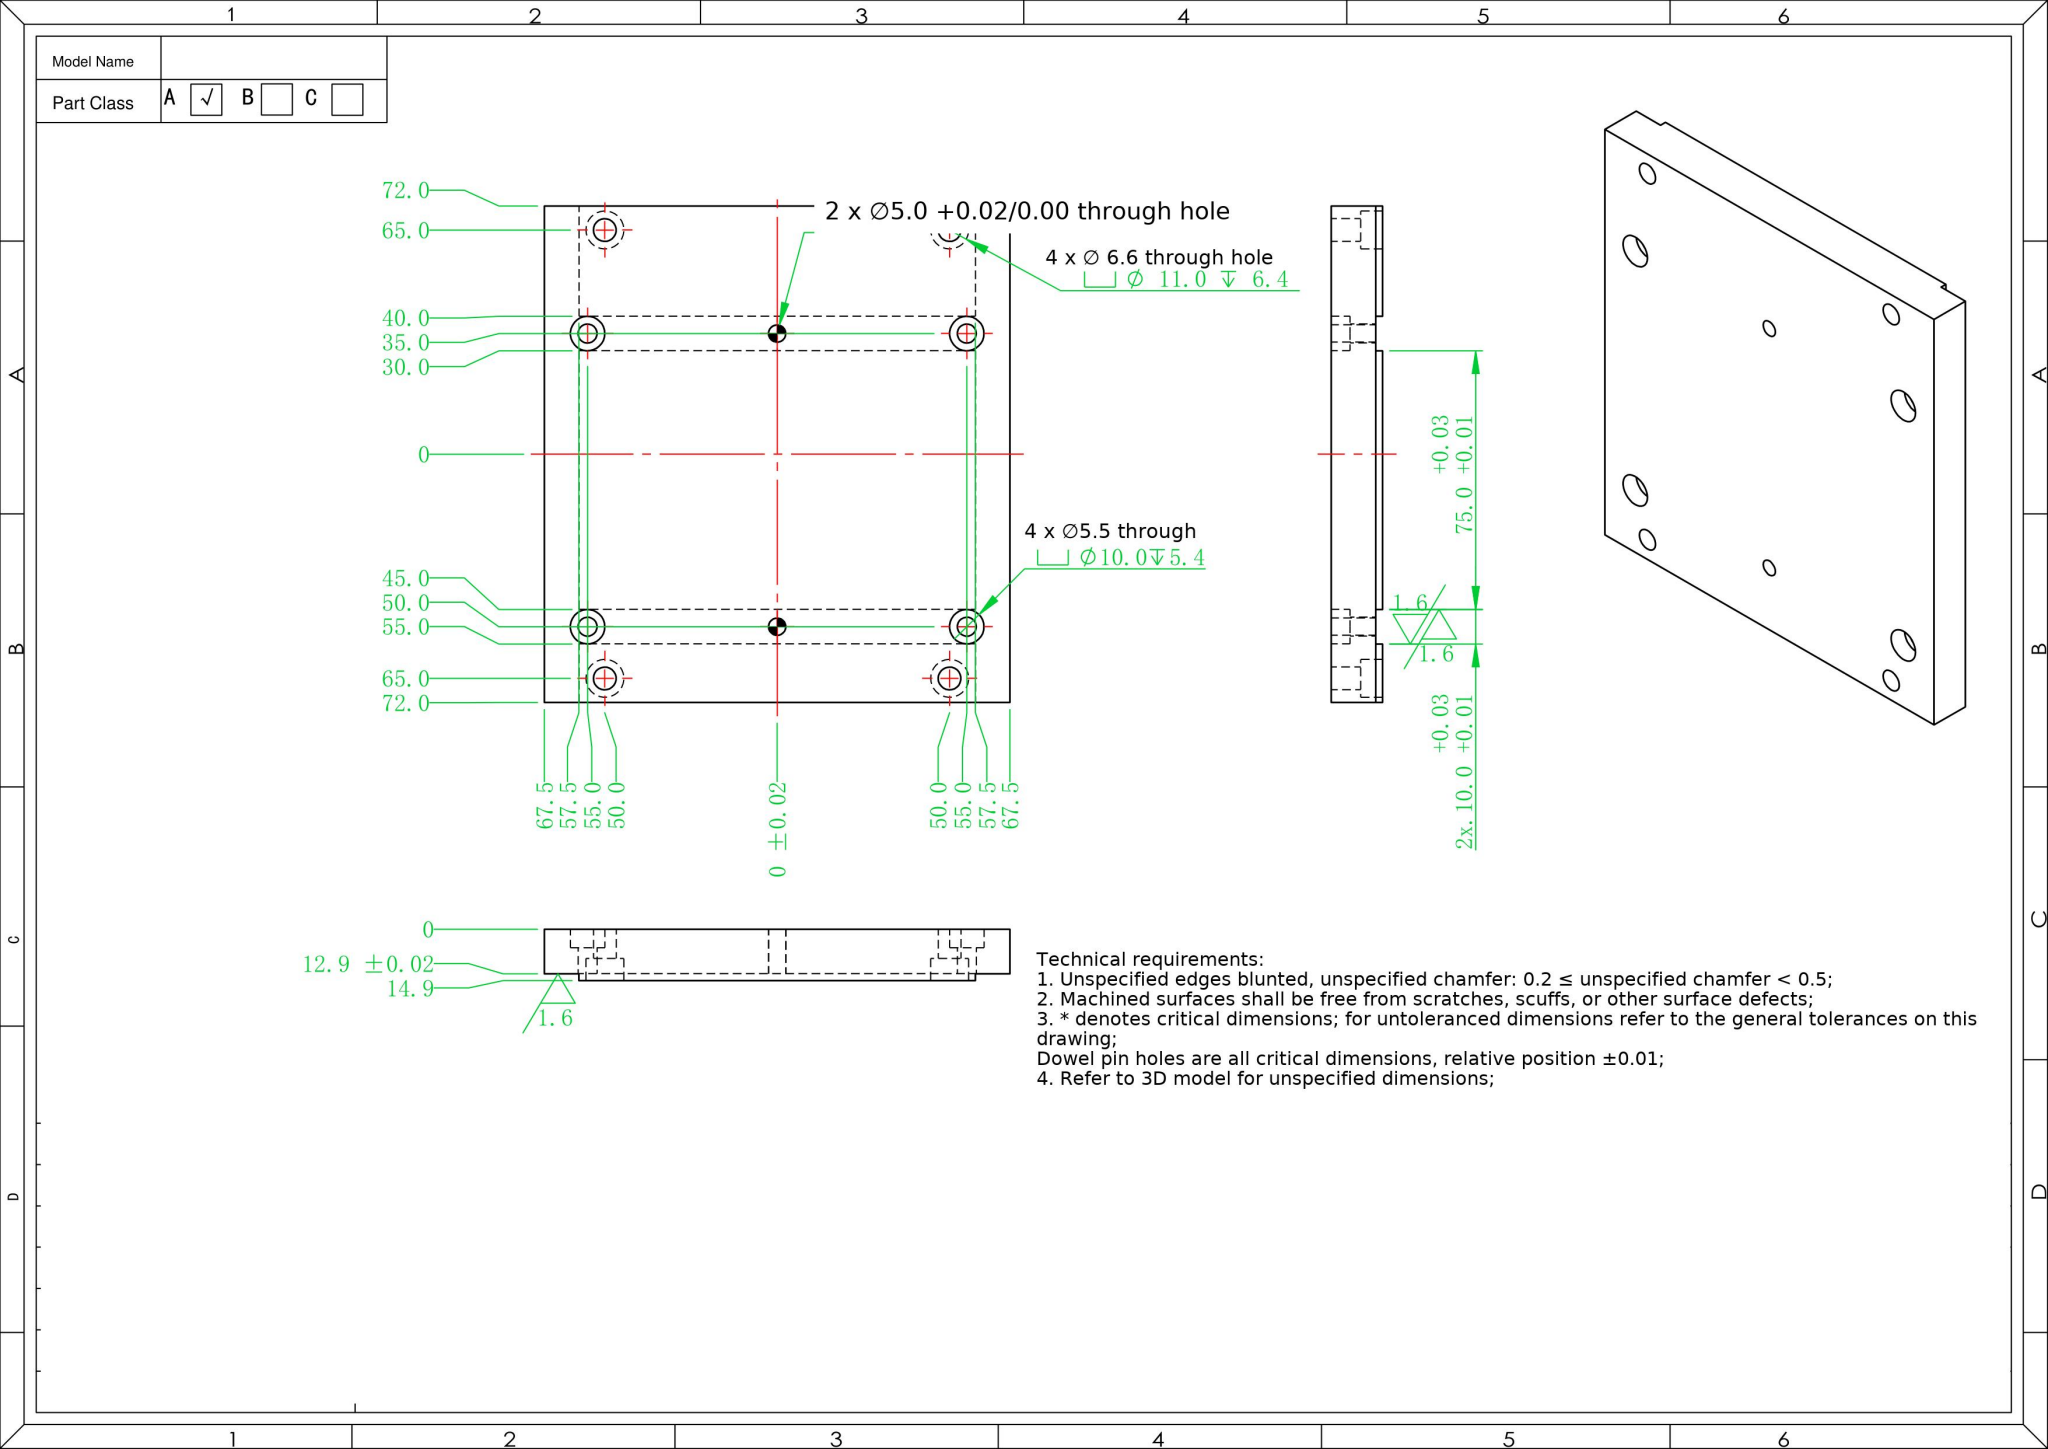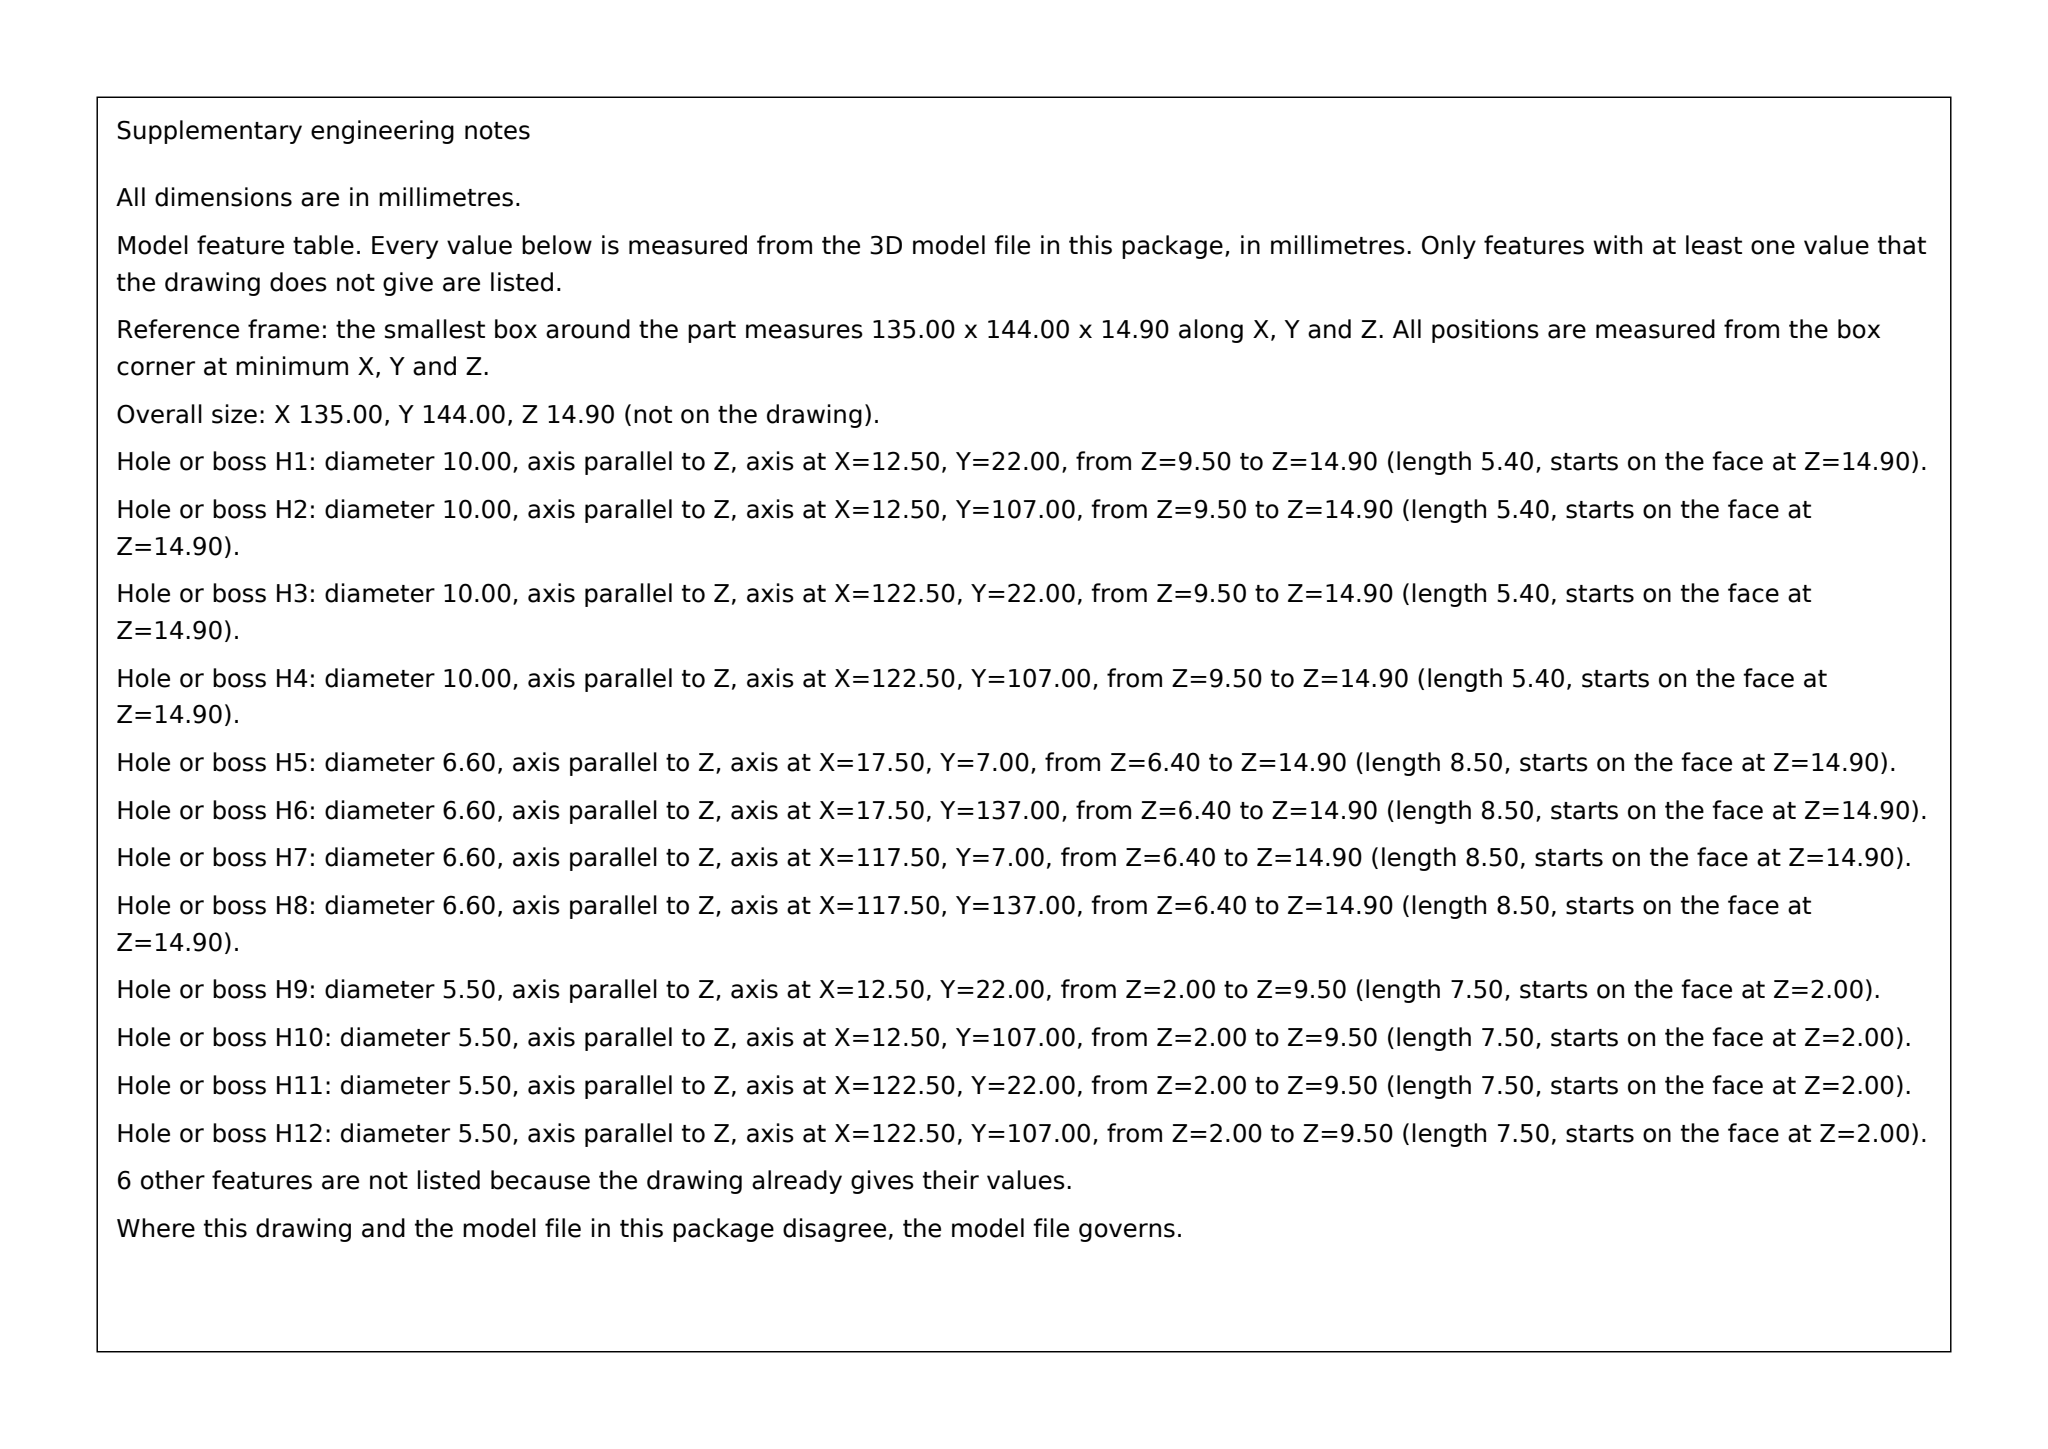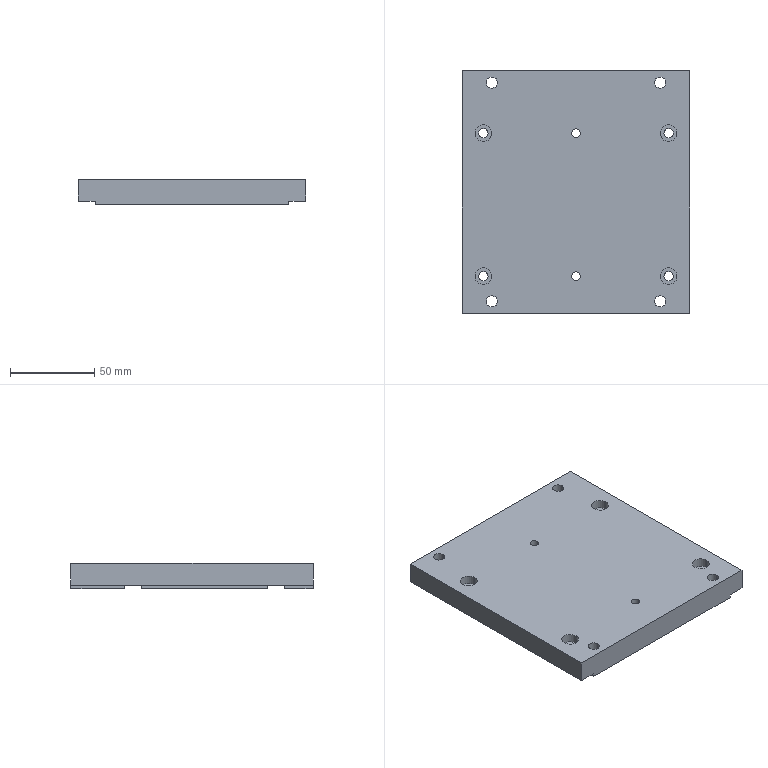Part | SolidWorks | mm | 1 solid | 63 faces | box 135 x 144 x 14.9 mm | volume 272784 mm3 | cylinder 36 | plane 27 | commonest cylinder face diameters 11 x8 6.6 x8 10 x8 5.5 x8 5 x4